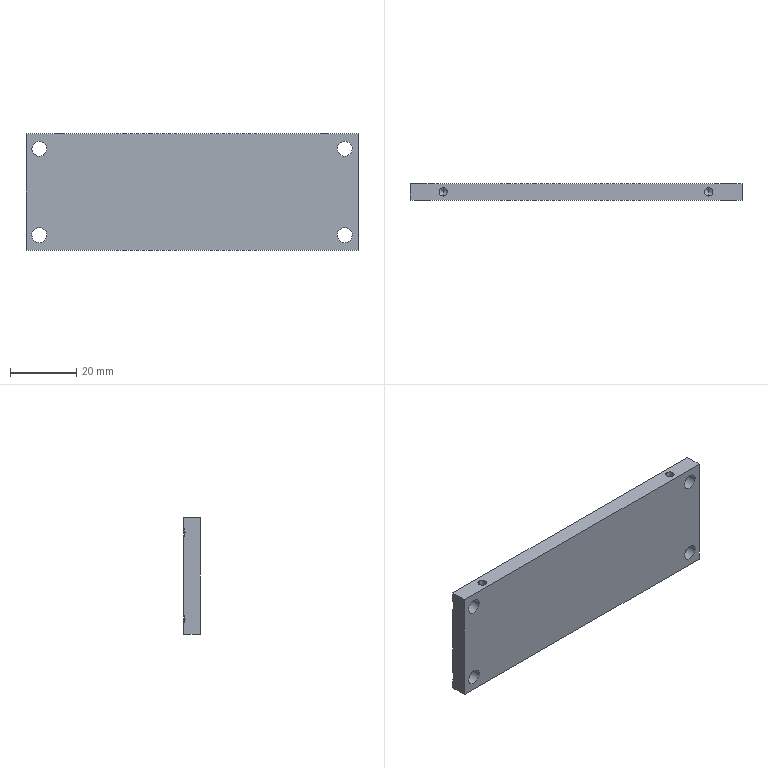CAM job | Mastercam | mm | 8 operations | part box 100 x 5 x 35
1. Facing | 24 - 100 平铣刀
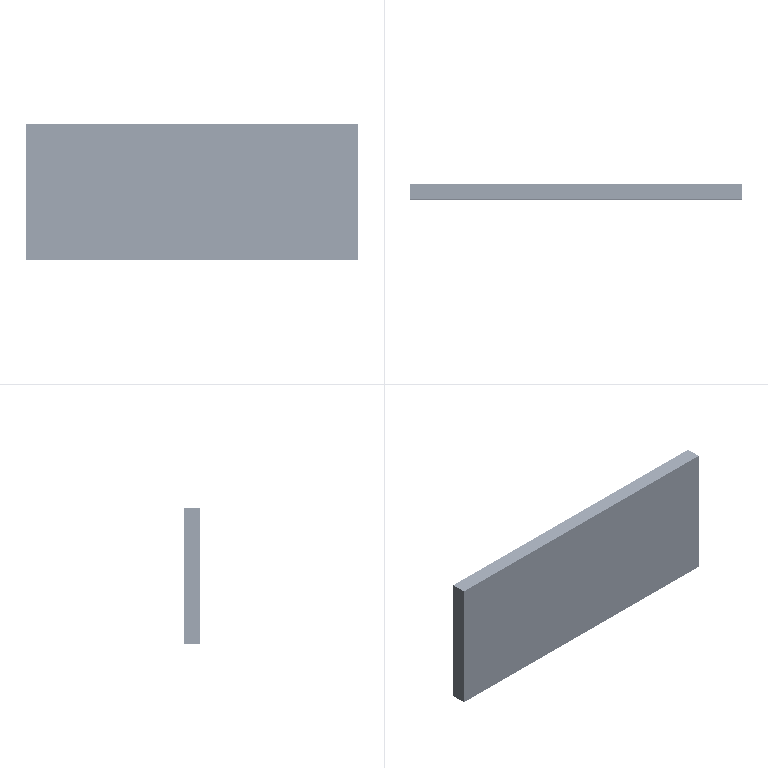2. Contour (Ramp) | 10 - 10 平铣刀
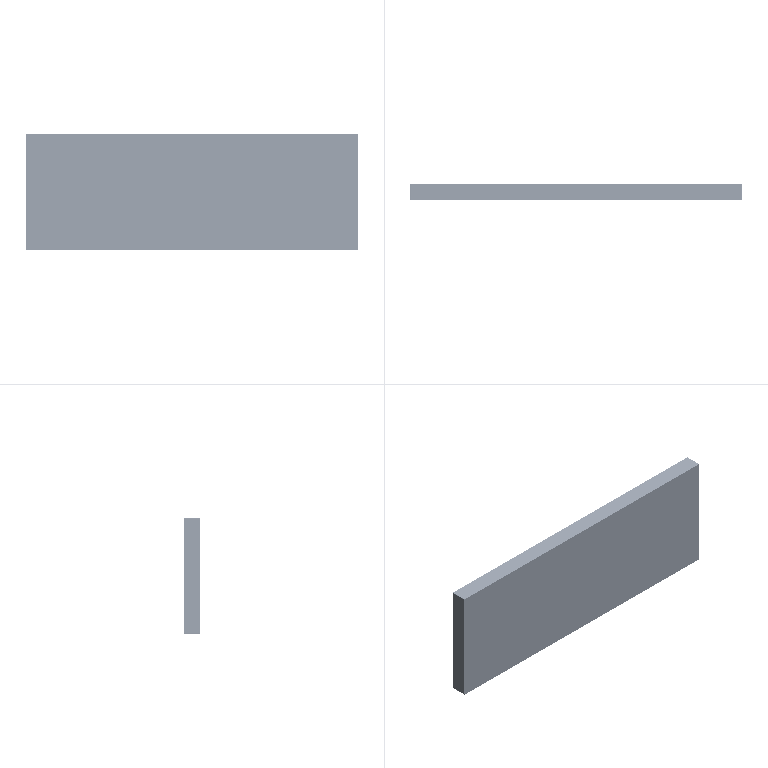3. Contour (2D) | 10 - 10 平铣刀
4. Contour (2D chamfer) | 7 - 4 倒角刀
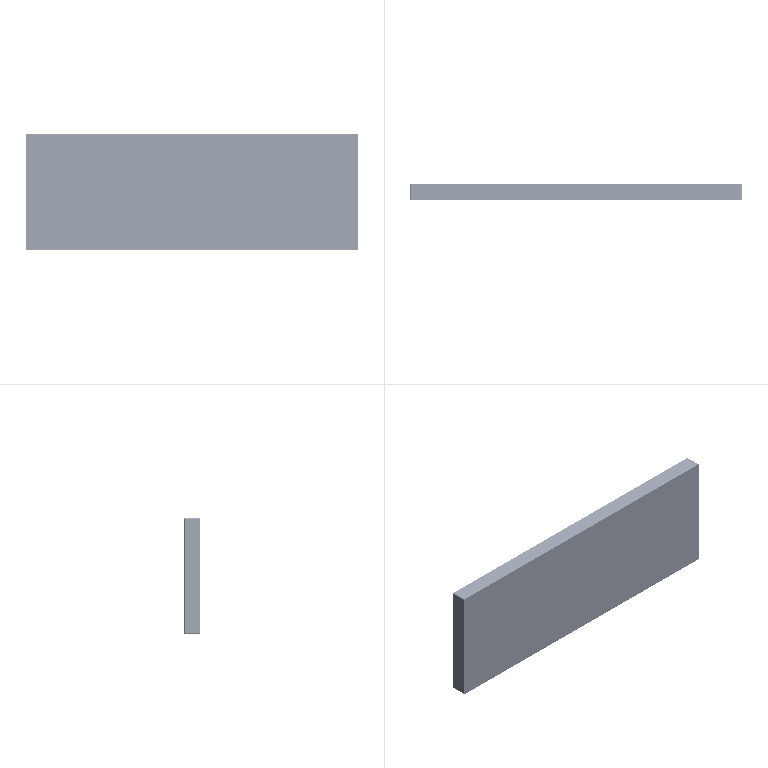5. Drill/Counterbore | 7 - 4 倒角刀
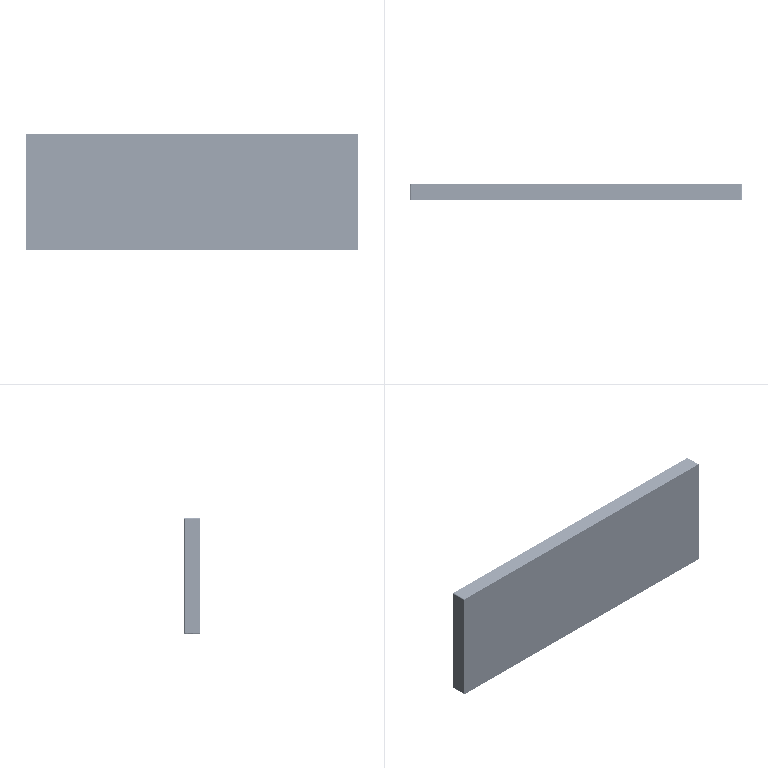6. Facing | 24 - 100 平铣刀
7. Contour (2D chamfer) | 7 - 4 倒角刀
8. Drill/Counterbore | 7 - 4 倒角刀